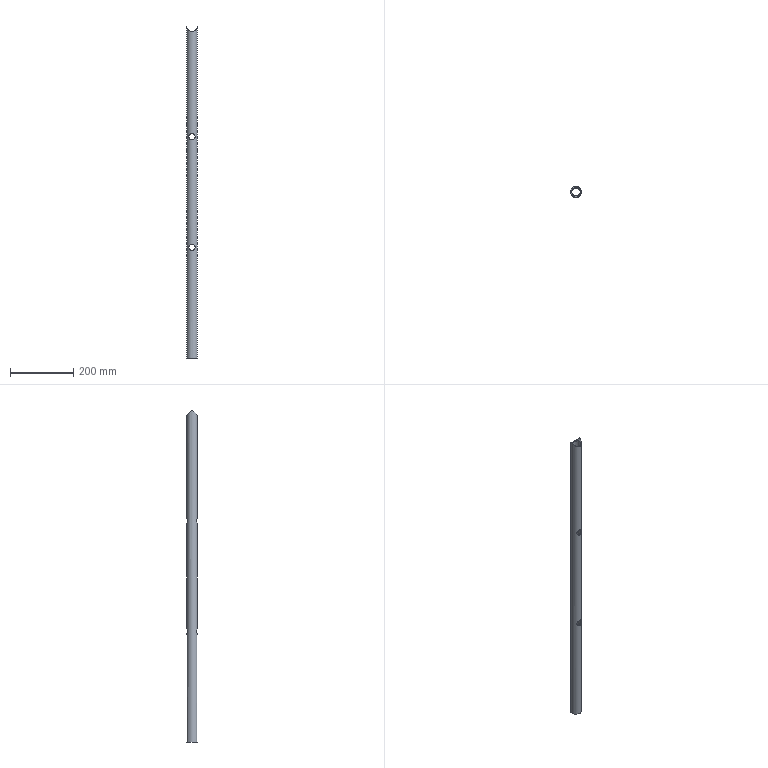Component | NX | 43_1_9 | 1 solid | 8 faces | volume 343237 mm3 | cylinder 7 | plane 1 | commonest cylinder face diameters 20 x4 34 x2 27 x1